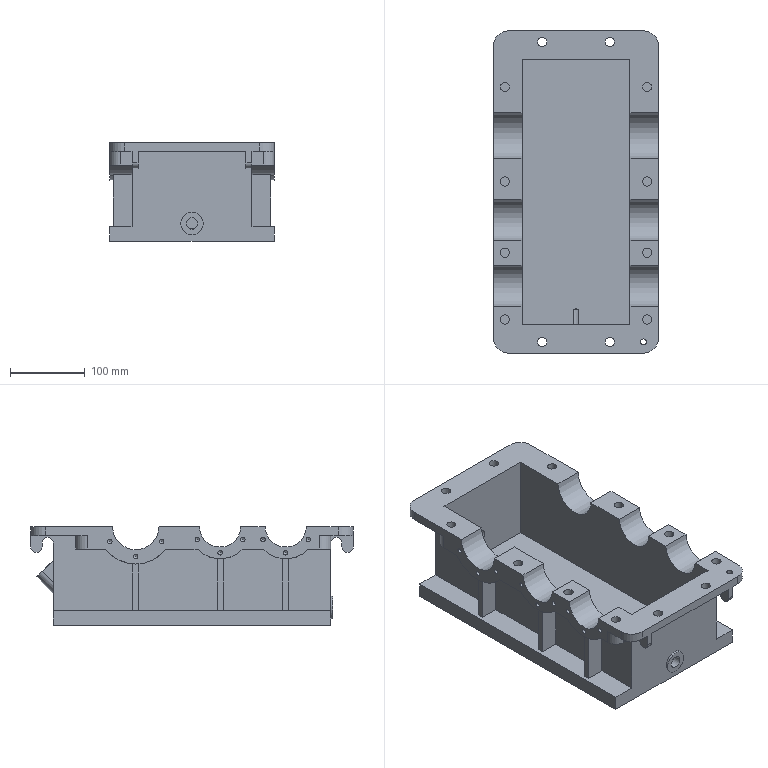Component | NX | XIANGTI | 1 solid | 162 faces | volume 3074507 mm3 | plane 79 | cylinder 64 | cone 19 | commonest cylinder face diameters 6 x18 12.5 x10 15 x9 30 x5 86 x4 55 x4 40 x4 100 x2